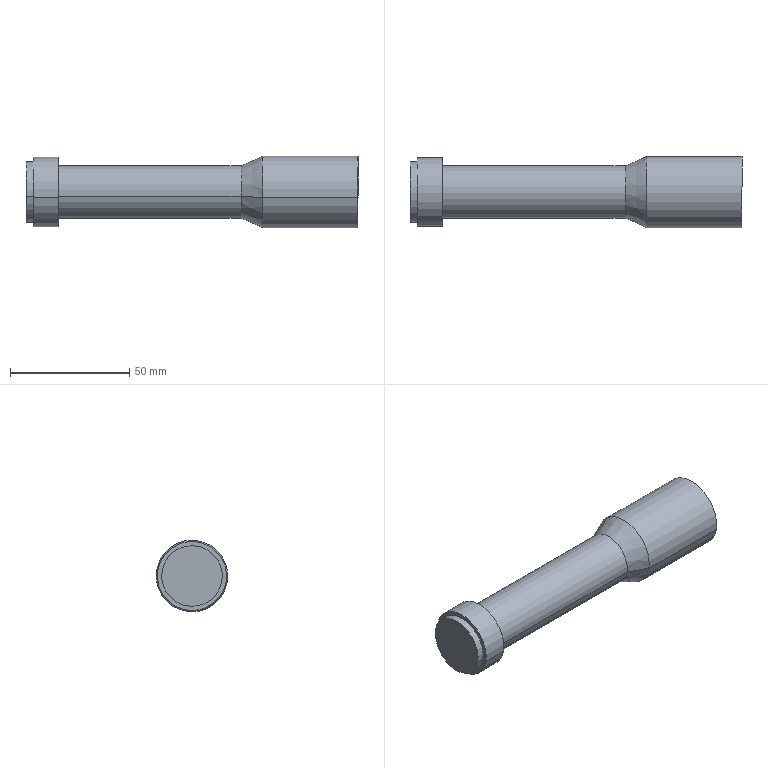Component | SolidWorks | ImagingSystem-1111-1_Lens-1111-2 | 1 solid | 14 faces | box 139.1 x 30 x 30 mm | volume 70664 mm3 | cylinder 8 | plane 4 | cone 2 | commonest cylinder face diameters 30 x2 25.4 x2 22 x2 29 x2
build123d program:
from build123d import *

# Parameters (mm, degrees)
SKETCH1_R           = 14.5
BOSS_EXTRUDE1_DEPTH = 13.5
SKETCH2_R           = 11
BOSS_EXTRUDE2_DEPTH = 76.6
SKETCH4_OUTSIDE_W   = 50.798
SKETCH4_OUTSIDE_H   = 50.798
SKETCH4_OUTSIDE_R   = 12.7
CUT_EXTRUDE1_DEPTH  = 3


with BuildPart() as part:
    # Sketch1 → Boss-Extrude1 (new body)
    with BuildSketch(Plane.XY):
        Circle(SKETCH1_R)
    extrude(amount=BOSS_EXTRUDE1_DEPTH)

    # Sketch2 → Boss-Extrude2 (add)
    with BuildSketch(Plane.XY.offset(13.5)):
        Circle(SKETCH2_R)
    extrude(amount=BOSS_EXTRUDE2_DEPTH)

    # Sketch4 outside → Cut-Extrude1 (cut)
    with BuildSketch(Plane(origin=(0, 0, 0), x_dir=(-1, 0, 0), z_dir=(0, 0, -1))):
        Rectangle(SKETCH4_OUTSIDE_W, SKETCH4_OUTSIDE_H)
        Circle(SKETCH4_OUTSIDE_R, mode=Mode.SUBTRACT)
    extrude(amount=-CUT_EXTRUDE1_DEPTH, mode=Mode.SUBTRACT)

    # Sketch3 → Revolve2 (revolve)
    with BuildSketch(Plane(origin=(0, 0, 0), x_dir=(0, 0, -1), z_dir=(1, 0, 0)), mode=Mode.PRIVATE) as revolve2_sk:
        Polygon((-90.1, 0), (-90.1, 11), (-99.1, 15), (-139.1, 15), (-139.1, 0), align=None)
    revolve(revolve2_sk.sketch.rotate(Axis((0, 0, 139.1), (0, 0, -1)), 90), axis=Axis((0, 0, 139.1), (0, 0, -1)))


solid = part.part

# Placed as in the assembly
solid = solid.moved(Location((31.194, -55, -75), (0, 90, 0)))
STEP:
#1=CARTESIAN_POINT('',(5.13,-1.582,-2.859));
#2=VERTEX_POINT('',#1);
#3=CARTESIAN_POINT('',(5.13,-2.748,-3.047));
#4=VERTEX_POINT('',#3);
#5=CARTESIAN_POINT('',(5.13,-2.165,-2.953));
#6=DIRECTION('',(1.,-0.,-0.));
#7=DIRECTION('',(0.,0.9873,0.1591));
#8=AXIS2_PLACEMENT_3D('',#5,#6,#7);
#9=CIRCLE('',#8,0.5906);
#10=EDGE_CURVE('',#2,#4,#9,.T.);
#11=ORIENTED_EDGE('',*,*,#10,.T.);
#12=CARTESIAN_POINT('',(6.704,-2.748,-3.047));
#13=VERTEX_POINT('',#12);
#14=CARTESIAN_POINT('',(6.704,-2.748,-3.047));
#15=DIRECTION('',(1.,-0.,-0.));
#16=VECTOR('',#15,39.37);
#17=LINE('',#14,#16);
#18=EDGE_CURVE('',#4,#13,#17,.T.);
#19=ORIENTED_EDGE('',*,*,#18,.T.);
#20=CARTESIAN_POINT('',(6.704,-1.582,-2.859));
#21=VERTEX_POINT('',#20);
#22=CARTESIAN_POINT('',(6.704,-2.165,-2.953));
#23=DIRECTION('',(1.,-0.,-0.));
#24=DIRECTION('',(0.,0.9873,0.1591));
#25=AXIS2_PLACEMENT_3D('',#22,#23,#24);
#26=CIRCLE('',#25,0.5906);
#27=EDGE_CURVE('',#21,#13,#26,.T.);
#28=ORIENTED_EDGE('',*,*,#27,.F.);
#29=CARTESIAN_POINT('',(6.704,-1.582,-2.859));
#30=DIRECTION('',(1.,-0.,-0.));
#31=VECTOR('',#30,39.37);
#32=LINE('',#29,#31);
#33=EDGE_CURVE('',#2,#21,#32,.T.);
#34=ORIENTED_EDGE('',*,*,#33,.F.);
#35=EDGE_LOOP('',(#11,#19,#28,#34));
#36=FACE_OUTER_BOUND('',#35,.T.);
#37=CARTESIAN_POINT('',(6.704,-2.165,-2.953));
#38=DIRECTION('',(1.,-0.,-0.));
#39=DIRECTION('',(0.,0.9873,0.1591));
#40=AXIS2_PLACEMENT_3D('',#37,#38,#39);
#41=CYLINDRICAL_SURFACE('',#40,0.5906);
#42=ADVANCED_FACE('',(#36),#41,.T.);
#43=CARTESIAN_POINT('',(4.775,-1.738,-2.884));
#44=VERTEX_POINT('',#43);
#45=CARTESIAN_POINT('',(4.775,-2.593,-3.022));
#46=VERTEX_POINT('',#45);
#47=CARTESIAN_POINT('',(4.775,-2.165,-2.953));
#48=DIRECTION('',(1.,-0.,-0.));
#49=DIRECTION('',(0.,0.9873,0.1591));
#50=AXIS2_PLACEMENT_3D('',#47,#48,#49);
#51=CIRCLE('',#50,0.4331);
#52=EDGE_CURVE('',#44,#46,#51,.T.);
#53=ORIENTED_EDGE('',*,*,#52,.T.);
#54=CARTESIAN_POINT('',(4.775,-2.593,-3.022));
#55=DIRECTION('',(0.9138,-0.401,-0.0646));
#56=VECTOR('',#55,39.37);
#57=LINE('',#54,#56);
#58=EDGE_CURVE('',#46,#4,#57,.T.);
#59=ORIENTED_EDGE('',*,*,#58,.T.);
#60=ORIENTED_EDGE('',*,*,#10,.F.);
#61=CARTESIAN_POINT('',(4.775,-1.738,-2.884));
#62=DIRECTION('',(0.9138,0.401,0.0646));
#63=VECTOR('',#62,39.37);
#64=LINE('',#61,#63);
#65=EDGE_CURVE('',#44,#2,#64,.T.);
#66=ORIENTED_EDGE('',*,*,#65,.F.);
#67=EDGE_LOOP('',(#53,#59,#60,#66));
#68=FACE_OUTER_BOUND('',#67,.T.);
#69=CARTESIAN_POINT('',(4.775,-2.165,-2.953));
#70=DIRECTION('',(1.,-0.,-0.));
#71=DIRECTION('',(0.,0.9873,0.1591));
#72=AXIS2_PLACEMENT_3D('',#69,#70,#71);
#73=CONICAL_SURFACE('',#72,0.4331,0.4182);
#74=ADVANCED_FACE('',(#68),#73,.T.);
#75=CARTESIAN_POINT('',(1.346,-2.659,-3.032));
#76=VERTEX_POINT('',#75);
#77=CARTESIAN_POINT('',(1.346,-1.672,-2.873));
#78=VERTEX_POINT('',#77);
#79=CARTESIAN_POINT('',(1.346,-2.165,-2.953));
#80=DIRECTION('',(-1.,0.,0.));
#81=DIRECTION('',(-0.,-0.9873,-0.1591));
#82=AXIS2_PLACEMENT_3D('',#79,#80,#81);
#83=CIRCLE('',#82,0.5);
#84=EDGE_CURVE('',#76,#78,#83,.T.);
#85=ORIENTED_EDGE('',*,*,#84,.T.);
#86=CARTESIAN_POINT('',(1.228,-1.672,-2.873));
#87=VERTEX_POINT('',#86);
#88=CARTESIAN_POINT('',(1.346,-1.672,-2.873));
#89=DIRECTION('',(-1.,0.,0.));
#90=VECTOR('',#89,39.37);
#91=LINE('',#88,#90);
#92=EDGE_CURVE('',#78,#87,#91,.T.);
#93=ORIENTED_EDGE('',*,*,#92,.T.);
#94=CARTESIAN_POINT('',(1.228,-2.659,-3.032));
#95=VERTEX_POINT('',#94);
#96=CARTESIAN_POINT('',(1.228,-2.165,-2.953));
#97=DIRECTION('',(-1.,0.,0.));
#98=DIRECTION('',(-0.,-0.9873,-0.1591));
#99=AXIS2_PLACEMENT_3D('',#96,#97,#98);
#100=CIRCLE('',#99,0.5);
#101=EDGE_CURVE('',#95,#87,#100,.T.);
#102=ORIENTED_EDGE('',*,*,#101,.F.);
#103=CARTESIAN_POINT('',(1.346,-2.659,-3.032));
#104=DIRECTION('',(-1.,0.,0.));
#105=VECTOR('',#104,39.37);
#106=LINE('',#103,#105);
#107=EDGE_CURVE('',#76,#95,#106,.T.);
#108=ORIENTED_EDGE('',*,*,#107,.F.);
#109=EDGE_LOOP('',(#85,#93,#102,#108));
#110=FACE_OUTER_BOUND('',#109,.T.);
#111=CARTESIAN_POINT('',(1.346,-2.165,-2.953));
#112=DIRECTION('',(-1.,0.,0.));
#113=DIRECTION('',(-0.,-0.9873,-0.1591));
#114=AXIS2_PLACEMENT_3D('',#111,#112,#113);
#115=CYLINDRICAL_SURFACE('',#114,0.5);
#116=ADVANCED_FACE('',(#110),#115,.T.);
#117=ORIENTED_EDGE('',*,*,#52,.F.);
#118=CARTESIAN_POINT('',(1.76,-1.738,-2.884));
#119=VERTEX_POINT('',#118);
#120=CARTESIAN_POINT('',(4.775,-1.738,-2.884));
#121=DIRECTION('',(-1.,0.,0.));
#122=VECTOR('',#121,39.37);
#123=LINE('',#120,#122);
#124=EDGE_CURVE('',#44,#119,#123,.T.);
#125=ORIENTED_EDGE('',*,*,#124,.T.);
#126=CARTESIAN_POINT('',(1.76,-2.593,-3.022));
#127=VERTEX_POINT('',#126);
#128=CARTESIAN_POINT('',(1.76,-2.165,-2.953));
#129=DIRECTION('',(1.,-0.,-0.));
#130=DIRECTION('',(0.,0.9873,0.1591));
#131=AXIS2_PLACEMENT_3D('',#128,#129,#130);
#132=CIRCLE('',#131,0.4331);
#133=EDGE_CURVE('',#119,#127,#132,.T.);
#134=ORIENTED_EDGE('',*,*,#133,.T.);
#135=CARTESIAN_POINT('',(4.775,-2.593,-3.022));
#136=DIRECTION('',(-1.,0.,0.));
#137=VECTOR('',#136,39.37);
#138=LINE('',#135,#137);
#139=EDGE_CURVE('',#46,#127,#138,.T.);
#140=ORIENTED_EDGE('',*,*,#139,.F.);
#141=EDGE_LOOP('',(#117,#125,#134,#140));
#142=FACE_OUTER_BOUND('',#141,.T.);
#143=CARTESIAN_POINT('',(4.775,-2.165,-2.953));
#144=DIRECTION('',(-1.,0.,0.));
#145=DIRECTION('',(-0.,-0.9873,-0.1591));
#146=AXIS2_PLACEMENT_3D('',#143,#144,#145);
#147=CYLINDRICAL_SURFACE('',#146,0.4331);
#148=ADVANCED_FACE('',(#142),#147,.T.);
#149=CARTESIAN_POINT('',(1.76,-1.602,-2.862));
#150=VERTEX_POINT('',#149);
#151=CARTESIAN_POINT('',(1.76,-2.729,-3.044));
#152=VERTEX_POINT('',#151);
#153=CARTESIAN_POINT('',(1.76,-2.165,-2.953));
#154=DIRECTION('',(1.,-0.,-0.));
#155=DIRECTION('',(0.,0.9873,0.1591));
#156=AXIS2_PLACEMENT_3D('',#153,#154,#155);
#157=CIRCLE('',#156,0.5709);
#158=EDGE_CURVE('',#150,#152,#157,.T.);
#159=ORIENTED_EDGE('',*,*,#158,.F.);
#160=CARTESIAN_POINT('',(1.346,-1.602,-2.862));
#161=VERTEX_POINT('',#160);
#162=CARTESIAN_POINT('',(1.76,-1.602,-2.862));
#163=DIRECTION('',(-1.,0.,0.));
#164=VECTOR('',#163,39.37);
#165=LINE('',#162,#164);
#166=EDGE_CURVE('',#150,#161,#165,.T.);
#167=ORIENTED_EDGE('',*,*,#166,.T.);
#168=CARTESIAN_POINT('',(1.346,-2.729,-3.044));
#169=VERTEX_POINT('',#168);
#170=CARTESIAN_POINT('',(1.346,-2.165,-2.953));
#171=DIRECTION('',(-1.,0.,0.));
#172=DIRECTION('',(-0.,-0.9873,-0.1591));
#173=AXIS2_PLACEMENT_3D('',#170,#171,#172);
#174=CIRCLE('',#173,0.5709);
#175=EDGE_CURVE('',#169,#161,#174,.T.);
#176=ORIENTED_EDGE('',*,*,#175,.F.);
#177=CARTESIAN_POINT('',(1.76,-2.729,-3.044));
#178=DIRECTION('',(-1.,0.,0.));
#179=VECTOR('',#178,39.37);
#180=LINE('',#177,#179);
#181=EDGE_CURVE('',#152,#169,#180,.T.);
#182=ORIENTED_EDGE('',*,*,#181,.F.);
#183=EDGE_LOOP('',(#159,#167,#176,#182));
#184=FACE_OUTER_BOUND('',#183,.T.);
#185=CARTESIAN_POINT('',(1.76,-2.165,-2.953));
#186=DIRECTION('',(-1.,0.,0.));
#187=DIRECTION('',(-0.,-0.9873,-0.1591));
#188=AXIS2_PLACEMENT_3D('',#185,#186,#187);
#189=CYLINDRICAL_SURFACE('',#188,0.5709);
#190=ADVANCED_FACE('',(#184),#189,.T.);
#191=ORIENTED_EDGE('',*,*,#166,.F.);
#192=CARTESIAN_POINT('',(1.76,-2.165,-2.953));
#193=DIRECTION('',(1.,-0.,-0.));
#194=DIRECTION('',(0.,0.9873,0.1591));
#195=AXIS2_PLACEMENT_3D('',#192,#193,#194);
#196=CIRCLE('',#195,0.5709);
#197=EDGE_CURVE('',#152,#150,#196,.T.);
#198=ORIENTED_EDGE('',*,*,#197,.F.);
#199=ORIENTED_EDGE('',*,*,#181,.T.);
#200=CARTESIAN_POINT('',(1.346,-2.165,-2.953));
#201=DIRECTION('',(-1.,0.,0.));
#202=DIRECTION('',(-0.,-0.9873,-0.1591));
#203=AXIS2_PLACEMENT_3D('',#200,#201,#202);
#204=CIRCLE('',#203,0.5709);
#205=EDGE_CURVE('',#161,#169,#204,.T.);
#206=ORIENTED_EDGE('',*,*,#205,.F.);
#207=EDGE_LOOP('',(#191,#198,#199,#206));
#208=FACE_OUTER_BOUND('',#207,.T.);
#209=CARTESIAN_POINT('',(1.76,-2.165,-2.953));
#210=DIRECTION('',(-1.,0.,0.));
#211=DIRECTION('',(-0.,-0.9873,-0.1591));
#212=AXIS2_PLACEMENT_3D('',#209,#210,#211);
#213=CYLINDRICAL_SURFACE('',#212,0.5709);
#214=ADVANCED_FACE('',(#208),#213,.T.);
#215=CARTESIAN_POINT('',(1.76,-2.165,-2.953));
#216=DIRECTION('',(1.,-0.,-0.));
#217=DIRECTION('',(0.,0.9873,0.1591));
#218=AXIS2_PLACEMENT_3D('',#215,#216,#217);
#219=CIRCLE('',#218,0.4331);
#220=EDGE_CURVE('',#127,#119,#219,.T.);
#221=ORIENTED_EDGE('',*,*,#220,.F.);
#222=ORIENTED_EDGE('',*,*,#133,.F.);
#223=EDGE_LOOP('',(#221,#222));
#224=FACE_BOUND('',#223,.T.);
#225=ORIENTED_EDGE('',*,*,#197,.T.);
#226=ORIENTED_EDGE('',*,*,#158,.T.);
#227=EDGE_LOOP('',(#225,#226));
#228=FACE_OUTER_BOUND('',#227,.T.);
#229=CARTESIAN_POINT('',(1.76,-2.165,-2.953));
#230=DIRECTION('',(1.,-0.,-0.));
#231=DIRECTION('',(0.,0.9873,0.1591));
#232=AXIS2_PLACEMENT_3D('',#229,#230,#231);
#233=PLANE('',#232);
#234=ADVANCED_FACE('',(#224,#228),#233,.T.);
#235=ORIENTED_EDGE('',*,*,#124,.F.);
#236=CARTESIAN_POINT('',(4.775,-2.165,-2.953));
#237=DIRECTION('',(1.,-0.,-0.));
#238=DIRECTION('',(0.,0.9873,0.1591));
#239=AXIS2_PLACEMENT_3D('',#236,#237,#238);
#240=CIRCLE('',#239,0.4331);
#241=EDGE_CURVE('',#46,#44,#240,.T.);
#242=ORIENTED_EDGE('',*,*,#241,.F.);
#243=ORIENTED_EDGE('',*,*,#139,.T.);
#244=ORIENTED_EDGE('',*,*,#220,.T.);
#245=EDGE_LOOP('',(#235,#242,#243,#244));
#246=FACE_OUTER_BOUND('',#245,.T.);
#247=CARTESIAN_POINT('',(4.775,-2.165,-2.953));
#248=DIRECTION('',(-1.,0.,0.));
#249=DIRECTION('',(-0.,-0.9873,-0.1591));
#250=AXIS2_PLACEMENT_3D('',#247,#248,#249);
#251=CYLINDRICAL_SURFACE('',#250,0.4331);
#252=ADVANCED_FACE('',(#246),#251,.T.);
#253=ORIENTED_EDGE('',*,*,#84,.F.);
#254=CARTESIAN_POINT('',(1.346,-2.165,-2.953));
#255=DIRECTION('',(-1.,0.,0.));
#256=DIRECTION('',(-0.,-0.9873,-0.1591));
#257=AXIS2_PLACEMENT_3D('',#254,#255,#256);
#258=CIRCLE('',#257,0.5);
#259=EDGE_CURVE('',#78,#76,#258,.T.);
#260=ORIENTED_EDGE('',*,*,#259,.F.);
#261=EDGE_LOOP('',(#253,#260));
#262=FACE_BOUND('',#261,.T.);
#263=ORIENTED_EDGE('',*,*,#175,.T.);
#264=ORIENTED_EDGE('',*,*,#205,.T.);
#265=EDGE_LOOP('',(#263,#264));
#266=FACE_OUTER_BOUND('',#265,.T.);
#267=CARTESIAN_POINT('',(1.346,-2.165,-2.953));
#268=DIRECTION('',(-1.,0.,0.));
#269=DIRECTION('',(-0.,-0.9873,-0.1591));
#270=AXIS2_PLACEMENT_3D('',#267,#268,#269);
#271=PLANE('',#270);
#272=ADVANCED_FACE('',(#262,#266),#271,.T.);
#273=ORIENTED_EDGE('',*,*,#92,.F.);
#274=ORIENTED_EDGE('',*,*,#259,.T.);
#275=ORIENTED_EDGE('',*,*,#107,.T.);
#276=CARTESIAN_POINT('',(1.228,-2.165,-2.953));
#277=DIRECTION('',(-1.,0.,0.));
#278=DIRECTION('',(-0.,-0.9873,-0.1591));
#279=AXIS2_PLACEMENT_3D('',#276,#277,#278);
#280=CIRCLE('',#279,0.5);
#281=EDGE_CURVE('',#87,#95,#280,.T.);
#282=ORIENTED_EDGE('',*,*,#281,.F.);
#283=EDGE_LOOP('',(#273,#274,#275,#282));
#284=FACE_OUTER_BOUND('',#283,.T.);
#285=CARTESIAN_POINT('',(1.346,-2.165,-2.953));
#286=DIRECTION('',(-1.,0.,0.));
#287=DIRECTION('',(-0.,-0.9873,-0.1591));
#288=AXIS2_PLACEMENT_3D('',#285,#286,#287);
#289=CYLINDRICAL_SURFACE('',#288,0.5);
#290=ADVANCED_FACE('',(#284),#289,.T.);
#291=ORIENTED_EDGE('',*,*,#101,.T.);
#292=ORIENTED_EDGE('',*,*,#281,.T.);
#293=EDGE_LOOP('',(#291,#292));
#294=FACE_OUTER_BOUND('',#293,.T.);
#295=CARTESIAN_POINT('',(1.228,-2.165,-2.953));
#296=DIRECTION('',(1.,-0.,-0.));
#297=DIRECTION('',(0.,0.9873,0.1591));
#298=AXIS2_PLACEMENT_3D('',#295,#296,#297);
#299=PLANE('',#298);
#300=ADVANCED_FACE('',(#294),#299,.F.);
#301=ORIENTED_EDGE('',*,*,#58,.F.);
#302=ORIENTED_EDGE('',*,*,#241,.T.);
#303=ORIENTED_EDGE('',*,*,#65,.T.);
#304=CARTESIAN_POINT('',(5.13,-2.165,-2.953));
#305=DIRECTION('',(1.,-0.,-0.));
#306=DIRECTION('',(0.,0.9873,0.1591));
#307=AXIS2_PLACEMENT_3D('',#304,#305,#306);
#308=CIRCLE('',#307,0.5906);
#309=EDGE_CURVE('',#4,#2,#308,.T.);
#310=ORIENTED_EDGE('',*,*,#309,.F.);
#311=EDGE_LOOP('',(#301,#302,#303,#310));
#312=FACE_OUTER_BOUND('',#311,.T.);
#313=CARTESIAN_POINT('',(4.775,-2.165,-2.953));
#314=DIRECTION('',(1.,-0.,-0.));
#315=DIRECTION('',(0.,0.9873,0.1591));
#316=AXIS2_PLACEMENT_3D('',#313,#314,#315);
#317=CONICAL_SURFACE('',#316,0.4331,0.4182);
#318=ADVANCED_FACE('',(#312),#317,.T.);
#319=ORIENTED_EDGE('',*,*,#18,.F.);
#320=ORIENTED_EDGE('',*,*,#309,.T.);
#321=ORIENTED_EDGE('',*,*,#33,.T.);
#322=CARTESIAN_POINT('',(6.704,-2.165,-2.953));
#323=DIRECTION('',(1.,-0.,-0.));
#324=DIRECTION('',(0.,0.9873,0.1591));
#325=AXIS2_PLACEMENT_3D('',#322,#323,#324);
#326=CIRCLE('',#325,0.5906);
#327=EDGE_CURVE('',#13,#21,#326,.T.);
#328=ORIENTED_EDGE('',*,*,#327,.F.);
#329=EDGE_LOOP('',(#319,#320,#321,#328));
#330=FACE_OUTER_BOUND('',#329,.T.);
#331=CARTESIAN_POINT('',(6.704,-2.165,-2.953));
#332=DIRECTION('',(1.,-0.,-0.));
#333=DIRECTION('',(0.,0.9873,0.1591));
#334=AXIS2_PLACEMENT_3D('',#331,#332,#333);
#335=CYLINDRICAL_SURFACE('',#334,0.5906);
#336=ADVANCED_FACE('',(#330),#335,.T.);
#337=ORIENTED_EDGE('',*,*,#27,.T.);
#338=ORIENTED_EDGE('',*,*,#327,.T.);
#339=EDGE_LOOP('',(#337,#338));
#340=FACE_OUTER_BOUND('',#339,.T.);
#341=CARTESIAN_POINT('',(6.704,-2.259,-2.37));
#342=DIRECTION('',(-1.,0.,0.));
#343=DIRECTION('',(-0.,-0.9873,-0.1591));
#344=AXIS2_PLACEMENT_3D('',#341,#342,#343);
#345=PLANE('',#344);
#346=ADVANCED_FACE('',(#340),#345,.F.);
#347=CLOSED_SHELL('',(#42,#74,#116,#148,#190,#214,#234,#252,#272,#290,#300,#318,#336,#346));
#348=MANIFOLD_SOLID_BREP('',#347);
#349=CARTESIAN_POINT('',(0.,0.,0.));
#350=DIRECTION('',(0.,0.,1.));
#351=DIRECTION('',(1.,0.,0.));
#352=AXIS2_PLACEMENT_3D('',#349,#350,#351);
#353=(LENGTH_UNIT()NAMED_UNIT(*)SI_UNIT($,.METRE.));
#354=LENGTH_MEASURE_WITH_UNIT(LENGTH_MEASURE(0.0254),#353);
#355=DIMENSIONAL_EXPONENTS(1.,0.,0.,0.,0.,0.,0.);
#356=(CONVERSION_BASED_UNIT('',#354)LENGTH_UNIT()NAMED_UNIT(#355));
#357=UNCERTAINTY_MEASURE_WITH_UNIT(LENGTH_MEASURE(0.00001),#356,'','');
#358=(NAMED_UNIT(*)PLANE_ANGLE_UNIT()SI_UNIT($,.RADIAN.));
#359=(NAMED_UNIT(*)SI_UNIT($,.STERADIAN.)SOLID_ANGLE_UNIT());
#360=(GEOMETRIC_REPRESENTATION_CONTEXT(3)GLOBAL_UNCERTAINTY_ASSIGNED_CONTEXT((#357))GLOBAL_UNIT_ASSIGNED_CONTEXT((#356,#358,#359))REPRESENTATION_CONTEXT('',''));
#361=ADVANCED_BREP_SHAPE_REPRESENTATION('',(#348,#352),#360);
#362=COLOUR_RGB('',0.7922,0.8196,0.9333);
#363=FILL_AREA_STYLE_COLOUR('',#362);
#364=FILL_AREA_STYLE('',(#363));
#365=SURFACE_STYLE_FILL_AREA(#364);
#366=SURFACE_SIDE_STYLE('',(#365));
#367=SURFACE_STYLE_USAGE(.BOTH.,#366);
#368=PRESENTATION_STYLE_ASSIGNMENT((#367));
#369=STYLED_ITEM('',(#368),#348);
#370=PRESENTATION_LAYER_ASSIGNMENT('','',(#369));
#371=(LENGTH_UNIT()NAMED_UNIT(*)SI_UNIT($,.METRE.));
#372=LENGTH_MEASURE_WITH_UNIT(LENGTH_MEASURE(0.0254),#371);
#373=DIMENSIONAL_EXPONENTS(1.,0.,0.,0.,0.,0.,0.);
#374=(CONVERSION_BASED_UNIT('',#372)LENGTH_UNIT()NAMED_UNIT(#373));
#375=UNCERTAINTY_MEASURE_WITH_UNIT(LENGTH_MEASURE(0.00001),#374,'','');
#376=(NAMED_UNIT(*)PLANE_ANGLE_UNIT()SI_UNIT($,.RADIAN.));
#377=(NAMED_UNIT(*)SI_UNIT($,.STERADIAN.)SOLID_ANGLE_UNIT());
#378=(GEOMETRIC_REPRESENTATION_CONTEXT(3)GLOBAL_UNCERTAINTY_ASSIGNED_CONTEXT((#375))GLOBAL_UNIT_ASSIGNED_CONTEXT((#374,#376,#377))REPRESENTATION_CONTEXT('',''));
#379=MECHANICAL_DESIGN_GEOMETRIC_PRESENTATION_REPRESENTATION('',(#369),#378);